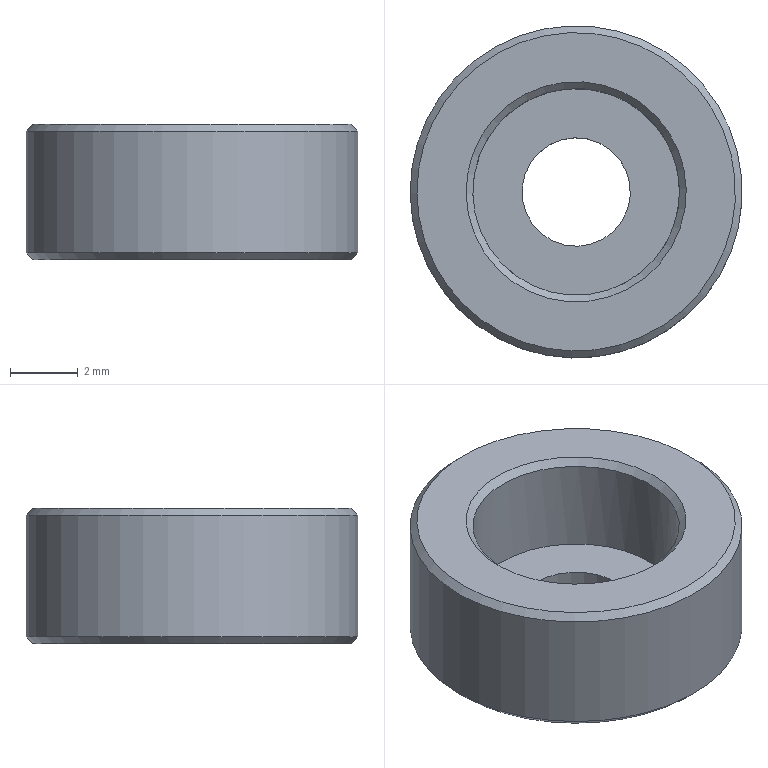Component | NX | DJZ_04_SPACER | 1 solid | 9 faces | box 9.8 x 9.8 x 4 mm | volume 204 mm3 | cylinder 3 | plane 3 | cone 3 | commonest cylinder face diameters 9.8 x1 6.1 x1 3.2 x1
STEP:
#1=CARTESIAN_POINT('',(0.,0.,0.));
#2=DIRECTION('',(0.,0.,1.));
#3=DIRECTION('',(1.,0.,0.));
#4=AXIS2_PLACEMENT_3D('',#1,#2,#3);
#5=CARTESIAN_POINT('',(4.526,1.877,3.7));
#6=VERTEX_POINT('',#5);
#7=CARTESIAN_POINT('',(0.,0.,3.7));
#8=DIRECTION('',(0.,0.,1.));
#9=DIRECTION('',(0.9237,0.383,0.));
#10=AXIS2_PLACEMENT_3D('',#7,#8,#9);
#11=CIRCLE('',#10,4.9);
#12=CARTESIAN_POINT('',(0.,0.,3.5));
#13=DIRECTION('',(0.,0.,1.));
#14=DIRECTION('',(-0.9237,-0.383,0.));
#15=AXIS2_PLACEMENT_3D('',#12,#13,#14);
#16=CYLINDRICAL_SURFACE('',#15,4.9);
#17=CARTESIAN_POINT('',(3.142,0.2));
#18=DIRECTION('',(1.,0.));
#19=VECTOR('',#18,1.);
#20=LINE('',#17,#19);
#21=(GEOMETRIC_REPRESENTATION_CONTEXT(2)PARAMETRIC_REPRESENTATION_CONTEXT()REPRESENTATION_CONTEXT('',''));
#22=DEFINITIONAL_REPRESENTATION('',(#20),#21);
#23=PCURVE('',#16,#22);
#24=CARTESIAN_POINT('',(0.,0.,3.5));
#25=DIRECTION('',(0.,0.,1.));
#26=DIRECTION('',(-0.9237,-0.383,0.));
#27=AXIS2_PLACEMENT_3D('',#24,#25,#26);
#28=CONICAL_SURFACE('',#27,4.7,0.7854);
#29=CARTESIAN_POINT('',(3.142,0.2));
#30=DIRECTION('',(1.,0.));
#31=VECTOR('',#30,1.);
#32=LINE('',#29,#31);
#33=(GEOMETRIC_REPRESENTATION_CONTEXT(2)PARAMETRIC_REPRESENTATION_CONTEXT()REPRESENTATION_CONTEXT('',''));
#34=DEFINITIONAL_REPRESENTATION('',(#32),#33);
#35=PCURVE('',#28,#34);
#36=SURFACE_CURVE('',#11,(#23,#35),.PCURVE_S1.);
#37=EDGE_CURVE('',#6,#6,#36,.T.);
#38=ORIENTED_EDGE('',*,*,#37,.T.);
#39=CARTESIAN_POINT('',(4.526,1.877,7.3));
#40=VERTEX_POINT('',#39);
#41=CARTESIAN_POINT('',(4.526,1.877,3.7));
#42=CARTESIAN_POINT('',(4.526,1.877,7.3));
#43=B_SPLINE_CURVE_WITH_KNOTS('',1,(#41,#42),.UNSPECIFIED.,.F.,.F.,(2,2),(0.2,3.8),.PIECEWISE_BEZIER_KNOTS.);
#44=CARTESIAN_POINT('',(9.425,0.));
#45=DIRECTION('',(0.,1.));
#46=VECTOR('',#45,1.);
#47=LINE('',#44,#46);
#48=(GEOMETRIC_REPRESENTATION_CONTEXT(2)PARAMETRIC_REPRESENTATION_CONTEXT()REPRESENTATION_CONTEXT('',''));
#49=DEFINITIONAL_REPRESENTATION('',(#47),#48);
#50=PCURVE('',#16,#49);
#51=CARTESIAN_POINT('',(3.142,0.));
#52=DIRECTION('',(0.,1.));
#53=VECTOR('',#52,1.);
#54=LINE('',#51,#53);
#55=(GEOMETRIC_REPRESENTATION_CONTEXT(2)PARAMETRIC_REPRESENTATION_CONTEXT()REPRESENTATION_CONTEXT('',''));
#56=DEFINITIONAL_REPRESENTATION('',(#54),#55);
#57=PCURVE('',#16,#56);
#58=SEAM_CURVE('',#43,(#50,#57),.PCURVE_S1.);
#59=EDGE_CURVE('',#6,#40,#58,.T.);
#60=ORIENTED_EDGE('',*,*,#59,.T.);
#61=CARTESIAN_POINT('',(0.,0.,7.3));
#62=DIRECTION('',(0.,0.,-1.));
#63=DIRECTION('',(0.9237,0.383,0.));
#64=AXIS2_PLACEMENT_3D('',#61,#62,#63);
#65=CIRCLE('',#64,4.9);
#66=CARTESIAN_POINT('',(9.425,3.8));
#67=DIRECTION('',(-1.,0.));
#68=VECTOR('',#67,1.);
#69=LINE('',#66,#68);
#70=(GEOMETRIC_REPRESENTATION_CONTEXT(2)PARAMETRIC_REPRESENTATION_CONTEXT()REPRESENTATION_CONTEXT('',''));
#71=DEFINITIONAL_REPRESENTATION('',(#69),#70);
#72=PCURVE('',#16,#71);
#73=CARTESIAN_POINT('',(0.,0.,7.3));
#74=DIRECTION('',(0.,0.,-1.));
#75=DIRECTION('',(0.9237,0.383,0.));
#76=AXIS2_PLACEMENT_3D('',#73,#74,#75);
#77=CONICAL_SURFACE('',#76,4.9,0.7854);
#78=CARTESIAN_POINT('',(0.,0.));
#79=DIRECTION('',(1.,-0.));
#80=VECTOR('',#79,1.);
#81=LINE('',#78,#80);
#82=(GEOMETRIC_REPRESENTATION_CONTEXT(2)PARAMETRIC_REPRESENTATION_CONTEXT()REPRESENTATION_CONTEXT('',''));
#83=DEFINITIONAL_REPRESENTATION('',(#81),#82);
#84=PCURVE('',#77,#83);
#85=SURFACE_CURVE('',#65,(#72,#84),.PCURVE_S1.);
#86=EDGE_CURVE('',#40,#40,#85,.T.);
#87=ORIENTED_EDGE('',*,*,#86,.T.);
#88=ORIENTED_EDGE('',*,*,#59,.F.);
#89=EDGE_LOOP('',(#38,#60,#87,#88));
#90=FACE_BOUND('',#89,.T.);
#91=ADVANCED_FACE('',(#90),#16,.T.);
#92=CARTESIAN_POINT('',(-2.817,-1.168,7.3));
#93=VERTEX_POINT('',#92);
#94=CARTESIAN_POINT('',(2.817,1.168,7.3));
#95=VERTEX_POINT('',#94);
#96=CARTESIAN_POINT('',(0.,0.,7.3));
#97=DIRECTION('',(0.,0.,1.));
#98=DIRECTION('',(0.9237,0.383,0.));
#99=AXIS2_PLACEMENT_3D('',#96,#97,#98);
#100=CIRCLE('',#99,3.05);
#101=CARTESIAN_POINT('',(0.,0.,3.5));
#102=DIRECTION('',(0.,0.,1.));
#103=DIRECTION('',(-0.9237,-0.383,0.));
#104=AXIS2_PLACEMENT_3D('',#101,#102,#103);
#105=CYLINDRICAL_SURFACE('',#104,3.05);
#106=CARTESIAN_POINT('',(-3.142,3.8));
#107=DIRECTION('',(1.,0.));
#108=VECTOR('',#107,1.);
#109=LINE('',#106,#108);
#110=(GEOMETRIC_REPRESENTATION_CONTEXT(2)PARAMETRIC_REPRESENTATION_CONTEXT()REPRESENTATION_CONTEXT('',''));
#111=DEFINITIONAL_REPRESENTATION('',(#109),#110);
#112=PCURVE('',#105,#111);
#113=CARTESIAN_POINT('',(0.,0.,7.5));
#114=DIRECTION('',(0.,0.,1.));
#115=DIRECTION('',(-0.9237,-0.383,0.));
#116=AXIS2_PLACEMENT_3D('',#113,#114,#115);
#117=CONICAL_SURFACE('',#116,3.25,0.7854);
#118=CARTESIAN_POINT('',(3.142,-0.2));
#119=DIRECTION('',(1.,0.));
#120=VECTOR('',#119,1.);
#121=LINE('',#118,#120);
#122=(GEOMETRIC_REPRESENTATION_CONTEXT(2)PARAMETRIC_REPRESENTATION_CONTEXT()REPRESENTATION_CONTEXT('',''));
#123=DEFINITIONAL_REPRESENTATION('',(#121),#122);
#124=PCURVE('',#117,#123);
#125=SURFACE_CURVE('',#100,(#112,#124),.PCURVE_S1.);
#126=EDGE_CURVE('',#93,#95,#125,.T.);
#127=ORIENTED_EDGE('',*,*,#126,.F.);
#128=CARTESIAN_POINT('',(-2.817,-1.168,4.5));
#129=VERTEX_POINT('',#128);
#130=CARTESIAN_POINT('',(-2.817,-1.168,4.5));
#131=CARTESIAN_POINT('',(-2.817,-1.168,7.3));
#132=B_SPLINE_CURVE_WITH_KNOTS('',1,(#130,#131),.UNSPECIFIED.,.F.,.F.,(2,2),(1.,3.8),.PIECEWISE_BEZIER_KNOTS.);
#133=CARTESIAN_POINT('',(0.,0.));
#134=DIRECTION('',(0.,1.));
#135=VECTOR('',#134,1.);
#136=LINE('',#133,#135);
#137=(GEOMETRIC_REPRESENTATION_CONTEXT(2)PARAMETRIC_REPRESENTATION_CONTEXT()REPRESENTATION_CONTEXT('',''));
#138=DEFINITIONAL_REPRESENTATION('',(#136),#137);
#139=PCURVE('',#105,#138);
#140=CARTESIAN_POINT('',(6.283,0.));
#141=DIRECTION('',(0.,1.));
#142=VECTOR('',#141,1.);
#143=LINE('',#140,#142);
#144=(GEOMETRIC_REPRESENTATION_CONTEXT(2)PARAMETRIC_REPRESENTATION_CONTEXT()REPRESENTATION_CONTEXT('',''));
#145=DEFINITIONAL_REPRESENTATION('',(#143),#144);
#146=PCURVE('',#105,#145);
#147=SEAM_CURVE('',#132,(#139,#146),.PCURVE_S1.);
#148=EDGE_CURVE('',#129,#93,#147,.T.);
#149=ORIENTED_EDGE('',*,*,#148,.F.);
#150=CARTESIAN_POINT('',(0.,0.,4.5));
#151=DIRECTION('',(0.,0.,1.));
#152=DIRECTION('',(-0.9237,-0.383,0.));
#153=AXIS2_PLACEMENT_3D('',#150,#151,#152);
#154=CIRCLE('',#153,3.05);
#155=CARTESIAN_POINT('',(0.,1.));
#156=DIRECTION('',(1.,0.));
#157=VECTOR('',#156,1.);
#158=LINE('',#155,#157);
#159=(GEOMETRIC_REPRESENTATION_CONTEXT(2)PARAMETRIC_REPRESENTATION_CONTEXT()REPRESENTATION_CONTEXT('',''));
#160=DEFINITIONAL_REPRESENTATION('',(#158),#159);
#161=PCURVE('',#105,#160);
#162=CARTESIAN_POINT('',(0.,0.,4.5));
#163=DIRECTION('',(0.,0.,1.));
#164=DIRECTION('',(-0.9237,-0.383,0.));
#165=AXIS2_PLACEMENT_3D('',#162,#163,#164);
#166=PLANE('',#165);
#167=CARTESIAN_POINT('',(0.,0.));
#168=DIRECTION('',(1.,0.));
#169=AXIS2_PLACEMENT_2D('',#167,#168);
#170=CIRCLE('',#169,3.05);
#171=(GEOMETRIC_REPRESENTATION_CONTEXT(2)PARAMETRIC_REPRESENTATION_CONTEXT()REPRESENTATION_CONTEXT('',''));
#172=DEFINITIONAL_REPRESENTATION('',(#170),#171);
#173=PCURVE('',#166,#172);
#174=SURFACE_CURVE('',#154,(#161,#173),.PCURVE_S1.);
#175=EDGE_CURVE('',#129,#129,#174,.T.);
#176=ORIENTED_EDGE('',*,*,#175,.T.);
#177=ORIENTED_EDGE('',*,*,#148,.T.);
#178=CARTESIAN_POINT('',(0.,0.,7.3));
#179=DIRECTION('',(0.,0.,1.));
#180=DIRECTION('',(0.9237,0.383,0.));
#181=AXIS2_PLACEMENT_3D('',#178,#179,#180);
#182=CIRCLE('',#181,3.05);
#183=CARTESIAN_POINT('',(3.142,3.8));
#184=DIRECTION('',(1.,0.));
#185=VECTOR('',#184,1.);
#186=LINE('',#183,#185);
#187=(GEOMETRIC_REPRESENTATION_CONTEXT(2)PARAMETRIC_REPRESENTATION_CONTEXT()REPRESENTATION_CONTEXT('',''));
#188=DEFINITIONAL_REPRESENTATION('',(#186),#187);
#189=PCURVE('',#105,#188);
#190=CARTESIAN_POINT('',(3.142,-0.2));
#191=DIRECTION('',(1.,-0.));
#192=VECTOR('',#191,1.);
#193=LINE('',#190,#192);
#194=(GEOMETRIC_REPRESENTATION_CONTEXT(2)PARAMETRIC_REPRESENTATION_CONTEXT()REPRESENTATION_CONTEXT('',''));
#195=DEFINITIONAL_REPRESENTATION('',(#193),#194);
#196=PCURVE('',#117,#195);
#197=SURFACE_CURVE('',#182,(#189,#196),.PCURVE_S1.);
#198=EDGE_CURVE('',#95,#93,#197,.T.);
#199=ORIENTED_EDGE('',*,*,#198,.F.);
#200=EDGE_LOOP('',(#127,#149,#176,#177,#199));
#201=FACE_BOUND('',#200,.F.);
#202=ADVANCED_FACE('',(#201),#105,.F.);
#203=CARTESIAN_POINT('',(4.342,1.8,3.5));
#204=VERTEX_POINT('',#203);
#205=CARTESIAN_POINT('',(0.,0.,3.5));
#206=DIRECTION('',(0.,0.,-1.));
#207=DIRECTION('',(0.9237,0.383,0.));
#208=AXIS2_PLACEMENT_3D('',#205,#206,#207);
#209=CIRCLE('',#208,4.7);
#210=CARTESIAN_POINT('',(0.,0.,3.5));
#211=DIRECTION('',(0.,0.,-1.));
#212=DIRECTION('',(0.9237,0.383,0.));
#213=AXIS2_PLACEMENT_3D('',#210,#211,#212);
#214=PLANE('',#213);
#215=CARTESIAN_POINT('',(0.,0.));
#216=DIRECTION('',(1.,0.));
#217=AXIS2_PLACEMENT_2D('',#215,#216);
#218=CIRCLE('',#217,4.7);
#219=(GEOMETRIC_REPRESENTATION_CONTEXT(2)PARAMETRIC_REPRESENTATION_CONTEXT()REPRESENTATION_CONTEXT('',''));
#220=DEFINITIONAL_REPRESENTATION('',(#218),#219);
#221=PCURVE('',#214,#220);
#222=CARTESIAN_POINT('',(9.425,0.));
#223=DIRECTION('',(-1.,0.));
#224=VECTOR('',#223,1.);
#225=LINE('',#222,#224);
#226=(GEOMETRIC_REPRESENTATION_CONTEXT(2)PARAMETRIC_REPRESENTATION_CONTEXT()REPRESENTATION_CONTEXT('',''));
#227=DEFINITIONAL_REPRESENTATION('',(#225),#226);
#228=PCURVE('',#28,#227);
#229=SURFACE_CURVE('',#209,(#221,#228),.PCURVE_S1.);
#230=EDGE_CURVE('',#204,#204,#229,.T.);
#231=ORIENTED_EDGE('',*,*,#230,.T.);
#232=EDGE_LOOP('',(#231));
#233=FACE_BOUND('',#232,.T.);
#234=CARTESIAN_POINT('',(1.478,0.6129,3.5));
#235=VERTEX_POINT('',#234);
#236=CARTESIAN_POINT('',(0.,0.,3.5));
#237=DIRECTION('',(0.,0.,1.));
#238=DIRECTION('',(0.9237,0.383,0.));
#239=AXIS2_PLACEMENT_3D('',#236,#237,#238);
#240=CIRCLE('',#239,1.6);
#241=CARTESIAN_POINT('',(1.6,0.));
#242=CARTESIAN_POINT('',(1.6,-2.771));
#243=CARTESIAN_POINT('',(-0.8,-1.386));
#244=CARTESIAN_POINT('',(-3.2,-0.));
#245=CARTESIAN_POINT('',(-0.8,1.386));
#246=CARTESIAN_POINT('',(1.6,2.771));
#247=CARTESIAN_POINT('',(1.6,0.));
#248=(BOUNDED_CURVE()B_SPLINE_CURVE(2,(#241,#242,#243,#244,#245,#246,#247),.UNSPECIFIED.,.T.,.F.)B_SPLINE_CURVE_WITH_KNOTS((1,2,2,2,2,1),(-2.094,0.,2.094,4.189,6.283,8.378),.UNSPECIFIED.)CURVE()GEOMETRIC_REPRESENTATION_ITEM()RATIONAL_B_SPLINE_CURVE((1.,0.5,1.,0.5,1.,0.5,1.))REPRESENTATION_ITEM(''));
#249=(GEOMETRIC_REPRESENTATION_CONTEXT(2)PARAMETRIC_REPRESENTATION_CONTEXT()REPRESENTATION_CONTEXT('',''));
#250=DEFINITIONAL_REPRESENTATION('',(#248),#249);
#251=PCURVE('',#214,#250);
#252=CARTESIAN_POINT('',(0.,0.,4.5));
#253=DIRECTION('',(0.,0.,-1.));
#254=DIRECTION('',(0.9237,0.383,0.));
#255=AXIS2_PLACEMENT_3D('',#252,#253,#254);
#256=CYLINDRICAL_SURFACE('',#255,1.6);
#257=CARTESIAN_POINT('',(6.283,1.));
#258=DIRECTION('',(-1.,0.));
#259=VECTOR('',#258,1.);
#260=LINE('',#257,#259);
#261=(GEOMETRIC_REPRESENTATION_CONTEXT(2)PARAMETRIC_REPRESENTATION_CONTEXT()REPRESENTATION_CONTEXT('',''));
#262=DEFINITIONAL_REPRESENTATION('',(#260),#261);
#263=PCURVE('',#256,#262);
#264=SURFACE_CURVE('',#240,(#251,#263),.PCURVE_S1.);
#265=EDGE_CURVE('',#235,#235,#264,.T.);
#266=ORIENTED_EDGE('',*,*,#265,.T.);
#267=EDGE_LOOP('',(#266));
#268=FACE_BOUND('',#267,.T.);
#269=ADVANCED_FACE('',(#233,#268),#214,.T.);
#270=CARTESIAN_POINT('',(3.002,1.245,7.5));
#271=VERTEX_POINT('',#270);
#272=CARTESIAN_POINT('',(0.,0.,7.5));
#273=DIRECTION('',(0.,0.,-1.));
#274=DIRECTION('',(0.9237,0.383,0.));
#275=AXIS2_PLACEMENT_3D('',#272,#273,#274);
#276=CIRCLE('',#275,3.25);
#277=CARTESIAN_POINT('',(0.,0.,7.5));
#278=DIRECTION('',(0.,0.,-1.));
#279=DIRECTION('',(0.9237,0.383,0.));
#280=AXIS2_PLACEMENT_3D('',#277,#278,#279);
#281=PLANE('',#280);
#282=CARTESIAN_POINT('',(0.,0.));
#283=DIRECTION('',(1.,0.));
#284=AXIS2_PLACEMENT_2D('',#282,#283);
#285=CIRCLE('',#284,3.25);
#286=(GEOMETRIC_REPRESENTATION_CONTEXT(2)PARAMETRIC_REPRESENTATION_CONTEXT()REPRESENTATION_CONTEXT('',''));
#287=DEFINITIONAL_REPRESENTATION('',(#285),#286);
#288=PCURVE('',#281,#287);
#289=CARTESIAN_POINT('',(9.425,0.));
#290=DIRECTION('',(-1.,-0.));
#291=VECTOR('',#290,1.);
#292=LINE('',#289,#291);
#293=(GEOMETRIC_REPRESENTATION_CONTEXT(2)PARAMETRIC_REPRESENTATION_CONTEXT()REPRESENTATION_CONTEXT('',''));
#294=DEFINITIONAL_REPRESENTATION('',(#292),#293);
#295=PCURVE('',#117,#294);
#296=SURFACE_CURVE('',#276,(#288,#295),.PCURVE_S1.);
#297=EDGE_CURVE('',#271,#271,#296,.T.);
#298=ORIENTED_EDGE('',*,*,#297,.T.);
#299=EDGE_LOOP('',(#298));
#300=FACE_BOUND('',#299,.T.);
#301=CARTESIAN_POINT('',(4.342,1.8,7.5));
#302=VERTEX_POINT('',#301);
#303=CARTESIAN_POINT('',(0.,0.,7.5));
#304=DIRECTION('',(0.,0.,1.));
#305=DIRECTION('',(0.9237,0.383,0.));
#306=AXIS2_PLACEMENT_3D('',#303,#304,#305);
#307=CIRCLE('',#306,4.7);
#308=CARTESIAN_POINT('',(4.7,0.));
#309=CARTESIAN_POINT('',(4.7,-8.141));
#310=CARTESIAN_POINT('',(-2.35,-4.07));
#311=CARTESIAN_POINT('',(-9.4,-0.));
#312=CARTESIAN_POINT('',(-2.35,4.07));
#313=CARTESIAN_POINT('',(4.7,8.141));
#314=CARTESIAN_POINT('',(4.7,0.));
#315=(BOUNDED_CURVE()B_SPLINE_CURVE(2,(#308,#309,#310,#311,#312,#313,#314),.UNSPECIFIED.,.T.,.F.)B_SPLINE_CURVE_WITH_KNOTS((1,2,2,2,2,1),(-2.094,0.,2.094,4.189,6.283,8.378),.UNSPECIFIED.)CURVE()GEOMETRIC_REPRESENTATION_ITEM()RATIONAL_B_SPLINE_CURVE((1.,0.5,1.,0.5,1.,0.5,1.))REPRESENTATION_ITEM(''));
#316=(GEOMETRIC_REPRESENTATION_CONTEXT(2)PARAMETRIC_REPRESENTATION_CONTEXT()REPRESENTATION_CONTEXT('',''));
#317=DEFINITIONAL_REPRESENTATION('',(#315),#316);
#318=PCURVE('',#281,#317);
#319=CARTESIAN_POINT('',(6.283,-0.2));
#320=DIRECTION('',(-1.,-0.));
#321=VECTOR('',#320,1.);
#322=LINE('',#319,#321);
#323=(GEOMETRIC_REPRESENTATION_CONTEXT(2)PARAMETRIC_REPRESENTATION_CONTEXT()REPRESENTATION_CONTEXT('',''));
#324=DEFINITIONAL_REPRESENTATION('',(#322),#323);
#325=PCURVE('',#77,#324);
#326=SURFACE_CURVE('',#307,(#318,#325),.PCURVE_S1.);
#327=EDGE_CURVE('',#302,#302,#326,.T.);
#328=ORIENTED_EDGE('',*,*,#327,.T.);
#329=EDGE_LOOP('',(#328));
#330=FACE_BOUND('',#329,.T.);
#331=ADVANCED_FACE('',(#300,#330),#281,.F.);
#332=CARTESIAN_POINT('',(1.478,0.6129,4.5));
#333=VERTEX_POINT('',#332);
#334=CARTESIAN_POINT('',(0.,0.,4.5));
#335=DIRECTION('',(0.,0.,1.));
#336=DIRECTION('',(0.9237,0.383,0.));
#337=AXIS2_PLACEMENT_3D('',#334,#335,#336);
#338=CIRCLE('',#337,1.6);
#339=CARTESIAN_POINT('',(0.,0.));
#340=DIRECTION('',(-1.,0.));
#341=AXIS2_PLACEMENT_2D('',#339,#340);
#342=CIRCLE('',#341,1.6);
#343=(GEOMETRIC_REPRESENTATION_CONTEXT(2)PARAMETRIC_REPRESENTATION_CONTEXT()REPRESENTATION_CONTEXT('',''));
#344=DEFINITIONAL_REPRESENTATION('',(#342),#343);
#345=PCURVE('',#166,#344);
#346=CARTESIAN_POINT('',(6.283,0.));
#347=DIRECTION('',(-1.,0.));
#348=VECTOR('',#347,1.);
#349=LINE('',#346,#348);
#350=(GEOMETRIC_REPRESENTATION_CONTEXT(2)PARAMETRIC_REPRESENTATION_CONTEXT()REPRESENTATION_CONTEXT('',''));
#351=DEFINITIONAL_REPRESENTATION('',(#349),#350);
#352=PCURVE('',#256,#351);
#353=SURFACE_CURVE('',#338,(#345,#352),.PCURVE_S1.);
#354=EDGE_CURVE('',#333,#333,#353,.T.);
#355=ORIENTED_EDGE('',*,*,#354,.F.);
#356=EDGE_LOOP('',(#355));
#357=FACE_BOUND('',#356,.T.);
#358=ORIENTED_EDGE('',*,*,#175,.T.);
#359=EDGE_LOOP('',(#358));
#360=FACE_BOUND('',#359,.T.);
#361=ADVANCED_FACE('',(#357,#360),#166,.T.);
#362=ORIENTED_EDGE('',*,*,#354,.F.);
#363=CARTESIAN_POINT('',(1.478,0.6129,4.5));
#364=CARTESIAN_POINT('',(1.478,0.6129,3.5));
#365=B_SPLINE_CURVE_WITH_KNOTS('',1,(#363,#364),.UNSPECIFIED.,.F.,.F.,(2,2),(0.,1.),.PIECEWISE_BEZIER_KNOTS.);
#366=CARTESIAN_POINT('',(6.283,0.));
#367=DIRECTION('',(0.,1.));
#368=VECTOR('',#367,1.);
#369=LINE('',#366,#368);
#370=(GEOMETRIC_REPRESENTATION_CONTEXT(2)PARAMETRIC_REPRESENTATION_CONTEXT()REPRESENTATION_CONTEXT('',''));
#371=DEFINITIONAL_REPRESENTATION('',(#369),#370);
#372=PCURVE('',#256,#371);
#373=CARTESIAN_POINT('',(0.,0.));
#374=DIRECTION('',(0.,1.));
#375=VECTOR('',#374,1.);
#376=LINE('',#373,#375);
#377=(GEOMETRIC_REPRESENTATION_CONTEXT(2)PARAMETRIC_REPRESENTATION_CONTEXT()REPRESENTATION_CONTEXT('',''));
#378=DEFINITIONAL_REPRESENTATION('',(#376),#377);
#379=PCURVE('',#256,#378);
#380=SEAM_CURVE('',#365,(#372,#379),.PCURVE_S1.);
#381=EDGE_CURVE('',#333,#235,#380,.T.);
#382=ORIENTED_EDGE('',*,*,#381,.T.);
#383=ORIENTED_EDGE('',*,*,#265,.T.);
#384=ORIENTED_EDGE('',*,*,#381,.F.);
#385=EDGE_LOOP('',(#362,#382,#383,#384));
#386=FACE_BOUND('',#385,.F.);
#387=ADVANCED_FACE('',(#386),#256,.F.);
#388=ORIENTED_EDGE('',*,*,#126,.T.);
#389=CARTESIAN_POINT('',(2.817,1.168,7.3));
#390=CARTESIAN_POINT('',(3.002,1.245,7.5));
#391=B_SPLINE_CURVE_WITH_KNOTS('',1,(#389,#390),.UNSPECIFIED.,.F.,.F.,(2,2),(-0.2828,0.),.PIECEWISE_BEZIER_KNOTS.);
#392=CARTESIAN_POINT('',(9.425,0.));
#393=DIRECTION('',(0.,1.));
#394=VECTOR('',#393,1.);
#395=LINE('',#392,#394);
#396=(GEOMETRIC_REPRESENTATION_CONTEXT(2)PARAMETRIC_REPRESENTATION_CONTEXT()REPRESENTATION_CONTEXT('',''));
#397=DEFINITIONAL_REPRESENTATION('',(#395),#396);
#398=PCURVE('',#117,#397);
#399=CARTESIAN_POINT('',(3.142,0.));
#400=DIRECTION('',(0.,1.));
#401=VECTOR('',#400,1.);
#402=LINE('',#399,#401);
#403=(GEOMETRIC_REPRESENTATION_CONTEXT(2)PARAMETRIC_REPRESENTATION_CONTEXT()REPRESENTATION_CONTEXT('',''));
#404=DEFINITIONAL_REPRESENTATION('',(#402),#403);
#405=PCURVE('',#117,#404);
#406=SEAM_CURVE('',#391,(#398,#405),.PCURVE_S1.);
#407=EDGE_CURVE('',#95,#271,#406,.T.);
#408=ORIENTED_EDGE('',*,*,#407,.T.);
#409=ORIENTED_EDGE('',*,*,#297,.T.);
#410=ORIENTED_EDGE('',*,*,#407,.F.);
#411=ORIENTED_EDGE('',*,*,#198,.T.);
#412=EDGE_LOOP('',(#388,#408,#409,#410,#411));
#413=FACE_BOUND('',#412,.F.);
#414=ADVANCED_FACE('',(#413),#117,.F.);
#415=ORIENTED_EDGE('',*,*,#37,.F.);
#416=CARTESIAN_POINT('',(4.342,1.8,3.5));
#417=CARTESIAN_POINT('',(4.526,1.877,3.7));
#418=B_SPLINE_CURVE_WITH_KNOTS('',1,(#416,#417),.UNSPECIFIED.,.F.,.F.,(2,2),(0.,0.2828),.PIECEWISE_BEZIER_KNOTS.);
#419=CARTESIAN_POINT('',(3.142,0.));
#420=DIRECTION('',(0.,1.));
#421=VECTOR('',#420,1.);
#422=LINE('',#419,#421);
#423=(GEOMETRIC_REPRESENTATION_CONTEXT(2)PARAMETRIC_REPRESENTATION_CONTEXT()REPRESENTATION_CONTEXT('',''));
#424=DEFINITIONAL_REPRESENTATION('',(#422),#423);
#425=PCURVE('',#28,#424);
#426=CARTESIAN_POINT('',(9.425,0.));
#427=DIRECTION('',(0.,1.));
#428=VECTOR('',#427,1.);
#429=LINE('',#426,#428);
#430=(GEOMETRIC_REPRESENTATION_CONTEXT(2)PARAMETRIC_REPRESENTATION_CONTEXT()REPRESENTATION_CONTEXT('',''));
#431=DEFINITIONAL_REPRESENTATION('',(#429),#430);
#432=PCURVE('',#28,#431);
#433=SEAM_CURVE('',#418,(#425,#432),.PCURVE_S1.);
#434=EDGE_CURVE('',#204,#6,#433,.T.);
#435=ORIENTED_EDGE('',*,*,#434,.F.);
#436=ORIENTED_EDGE('',*,*,#230,.F.);
#437=ORIENTED_EDGE('',*,*,#434,.T.);
#438=EDGE_LOOP('',(#415,#435,#436,#437));
#439=FACE_BOUND('',#438,.T.);
#440=ADVANCED_FACE('',(#439),#28,.T.);
#441=ORIENTED_EDGE('',*,*,#327,.F.);
#442=CARTESIAN_POINT('',(4.342,1.8,7.5));
#443=CARTESIAN_POINT('',(4.526,1.877,7.3));
#444=B_SPLINE_CURVE_WITH_KNOTS('',1,(#442,#443),.UNSPECIFIED.,.F.,.F.,(2,2),(-0.2828,0.),.PIECEWISE_BEZIER_KNOTS.);
#445=CARTESIAN_POINT('',(6.283,0.));
#446=DIRECTION('',(0.,1.));
#447=VECTOR('',#446,1.);
#448=LINE('',#445,#447);
#449=(GEOMETRIC_REPRESENTATION_CONTEXT(2)PARAMETRIC_REPRESENTATION_CONTEXT()REPRESENTATION_CONTEXT('',''));
#450=DEFINITIONAL_REPRESENTATION('',(#448),#449);
#451=PCURVE('',#77,#450);
#452=CARTESIAN_POINT('',(0.,0.));
#453=DIRECTION('',(0.,1.));
#454=VECTOR('',#453,1.);
#455=LINE('',#452,#454);
#456=(GEOMETRIC_REPRESENTATION_CONTEXT(2)PARAMETRIC_REPRESENTATION_CONTEXT()REPRESENTATION_CONTEXT('',''));
#457=DEFINITIONAL_REPRESENTATION('',(#455),#456);
#458=PCURVE('',#77,#457);
#459=SEAM_CURVE('',#444,(#451,#458),.PCURVE_S1.);
#460=EDGE_CURVE('',#302,#40,#459,.T.);
#461=ORIENTED_EDGE('',*,*,#460,.T.);
#462=ORIENTED_EDGE('',*,*,#86,.F.);
#463=ORIENTED_EDGE('',*,*,#460,.F.);
#464=EDGE_LOOP('',(#441,#461,#462,#463));
#465=FACE_BOUND('',#464,.T.);
#466=ADVANCED_FACE('',(#465),#77,.T.);
#467=CLOSED_SHELL('',(#91,#202,#269,#331,#361,#387,#414,#440,#466));
#468=MANIFOLD_SOLID_BREP('',#467);
#469=(LENGTH_UNIT()NAMED_UNIT(*)SI_UNIT(.MILLI.,.METRE.));
#470=UNCERTAINTY_MEASURE_WITH_UNIT(LENGTH_MEASURE(0.00001),#469,'','');
#471=(NAMED_UNIT(*)PLANE_ANGLE_UNIT()SI_UNIT($,.RADIAN.));
#472=(NAMED_UNIT(*)SI_UNIT($,.STERADIAN.)SOLID_ANGLE_UNIT());
#473=(GEOMETRIC_REPRESENTATION_CONTEXT(3)GLOBAL_UNCERTAINTY_ASSIGNED_CONTEXT((#470))GLOBAL_UNIT_ASSIGNED_CONTEXT((#469,#471,#472))REPRESENTATION_CONTEXT('',''));
#474=ADVANCED_BREP_SHAPE_REPRESENTATION('',(#4,#468),#473);